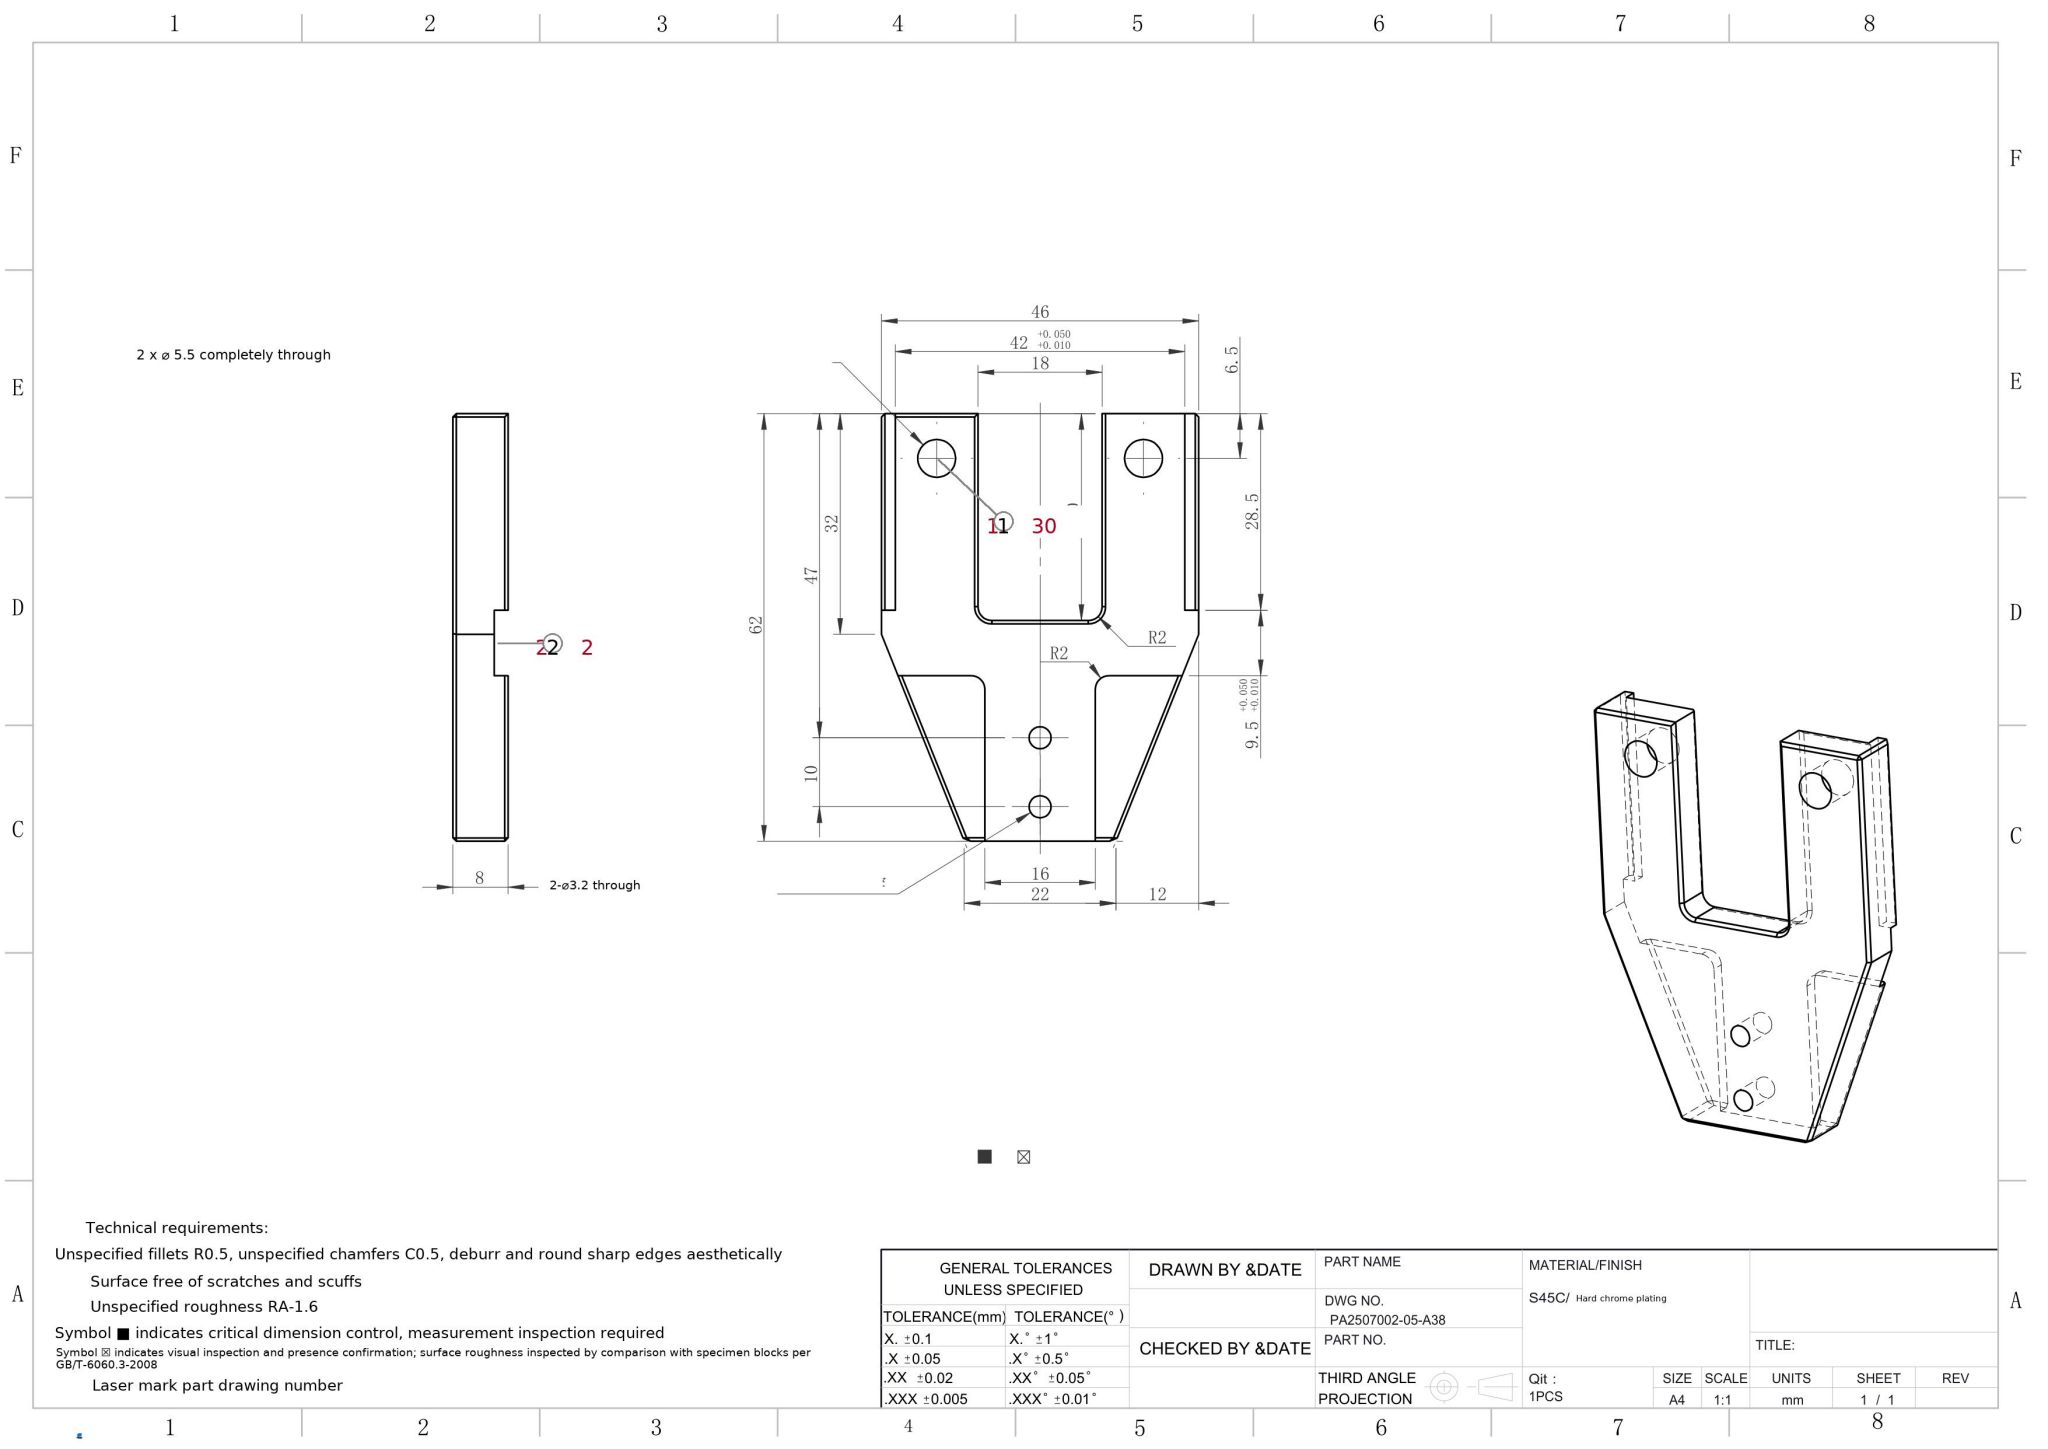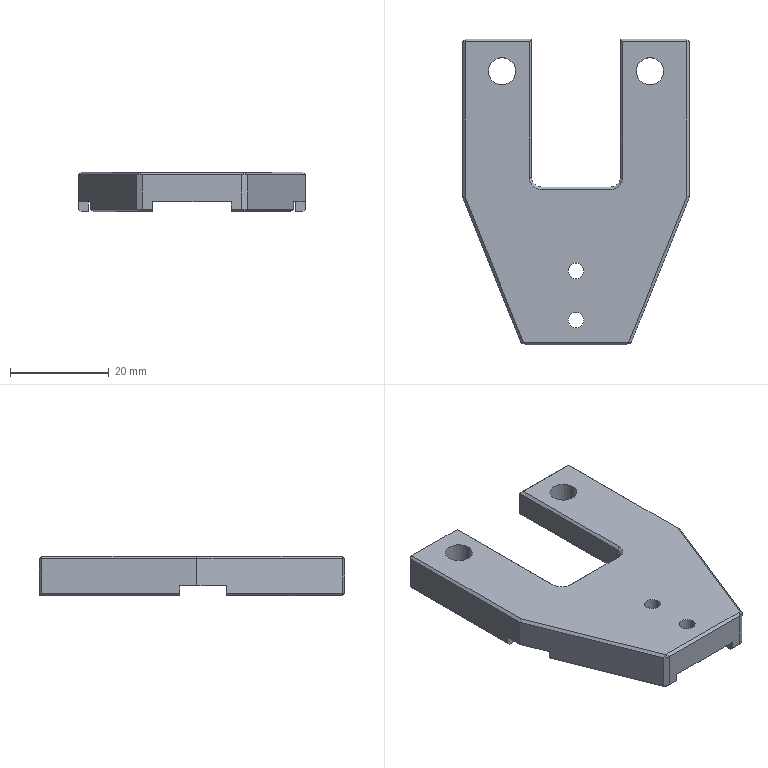Part | SolidWorks | mm | material S45C/ Hard chrome plating | 1 solid | 70 faces | box 46 x 62 x 8 mm | volume 12252 mm3 | plane 54 | cylinder 12 | cone 4 | commonest cylinder face diameters 3.2 x4 5.5 x4 4 x4